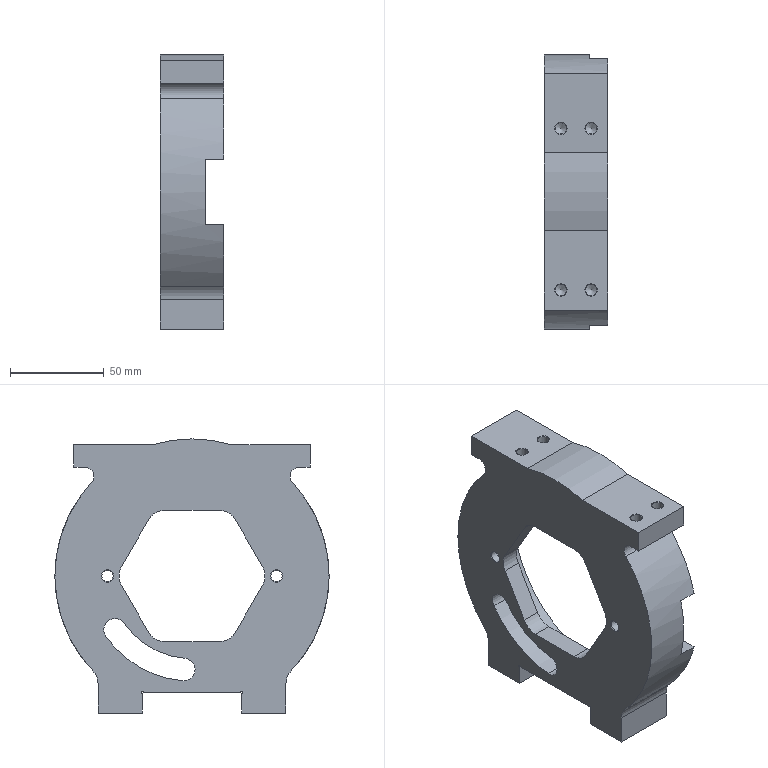Component | NX | HOUSING | 1 solid | 90 faces | volume 246977 mm3 | cylinder 35 | plane 31 | cone 24 | commonest cylinder face diameters 6 x12 20 x8 146 x3 130 x3 10 x2 1 x2 12 x2 120 x1